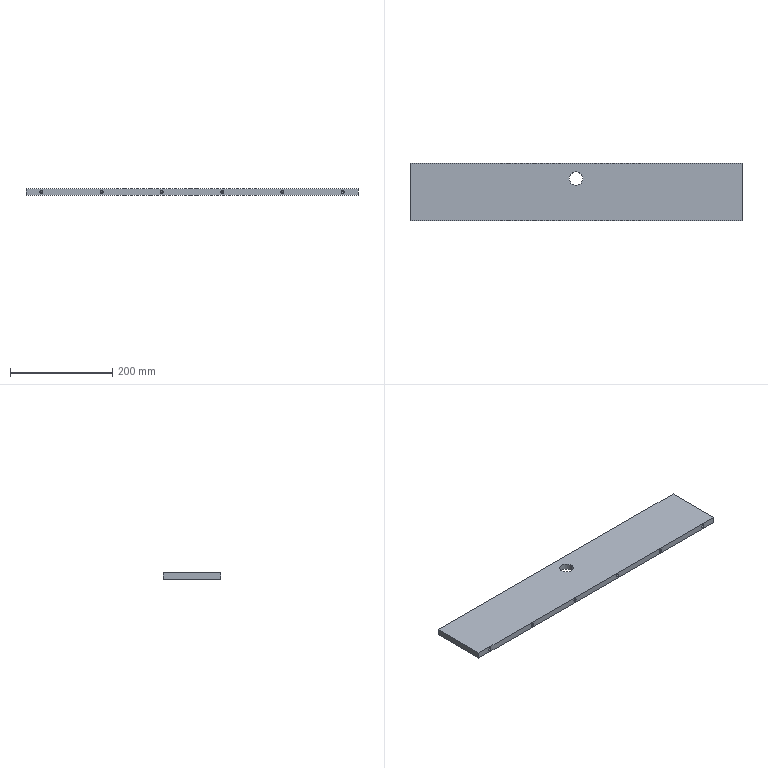CAM job | Mastercam | mm | 8 operations | part box 650 x 112.6 x 12
1. Contour (Ramp) | 10 - 10 平铣刀
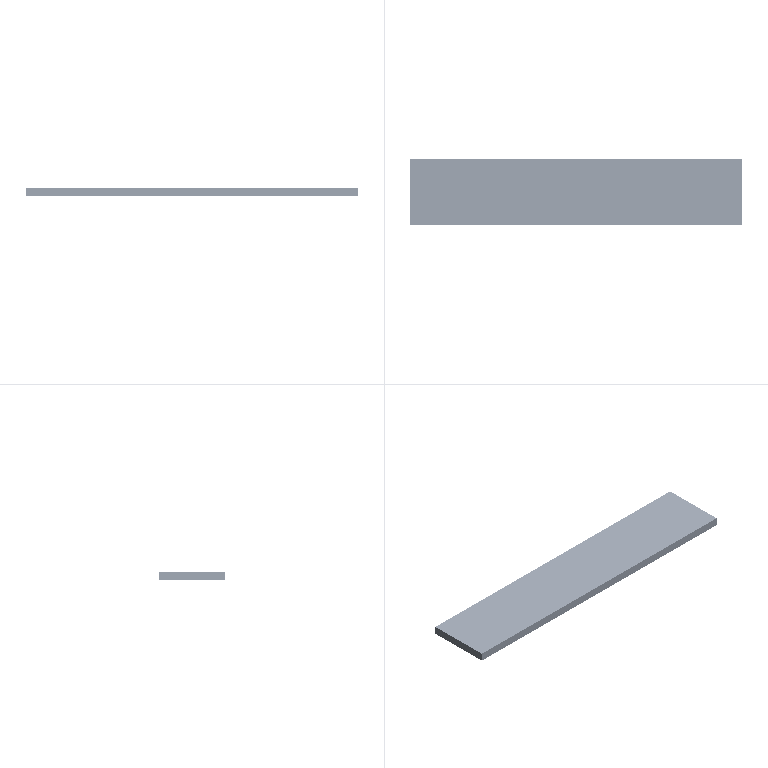2. Contour (Ramp) | 10 - 10 平铣刀
3. Contour (2D) | 10 - 10 平铣刀
4. Contour (2D) | 10 - 10 平铣刀
5. Contour (Ramp) | 10 - 10 平铣刀
6. Contour (2D) | 10 - 10 平铣刀
7. Drill/Counterbore | 7 - 4 倒角刀
8. Peck Drill | 1 - 5.1 钻头